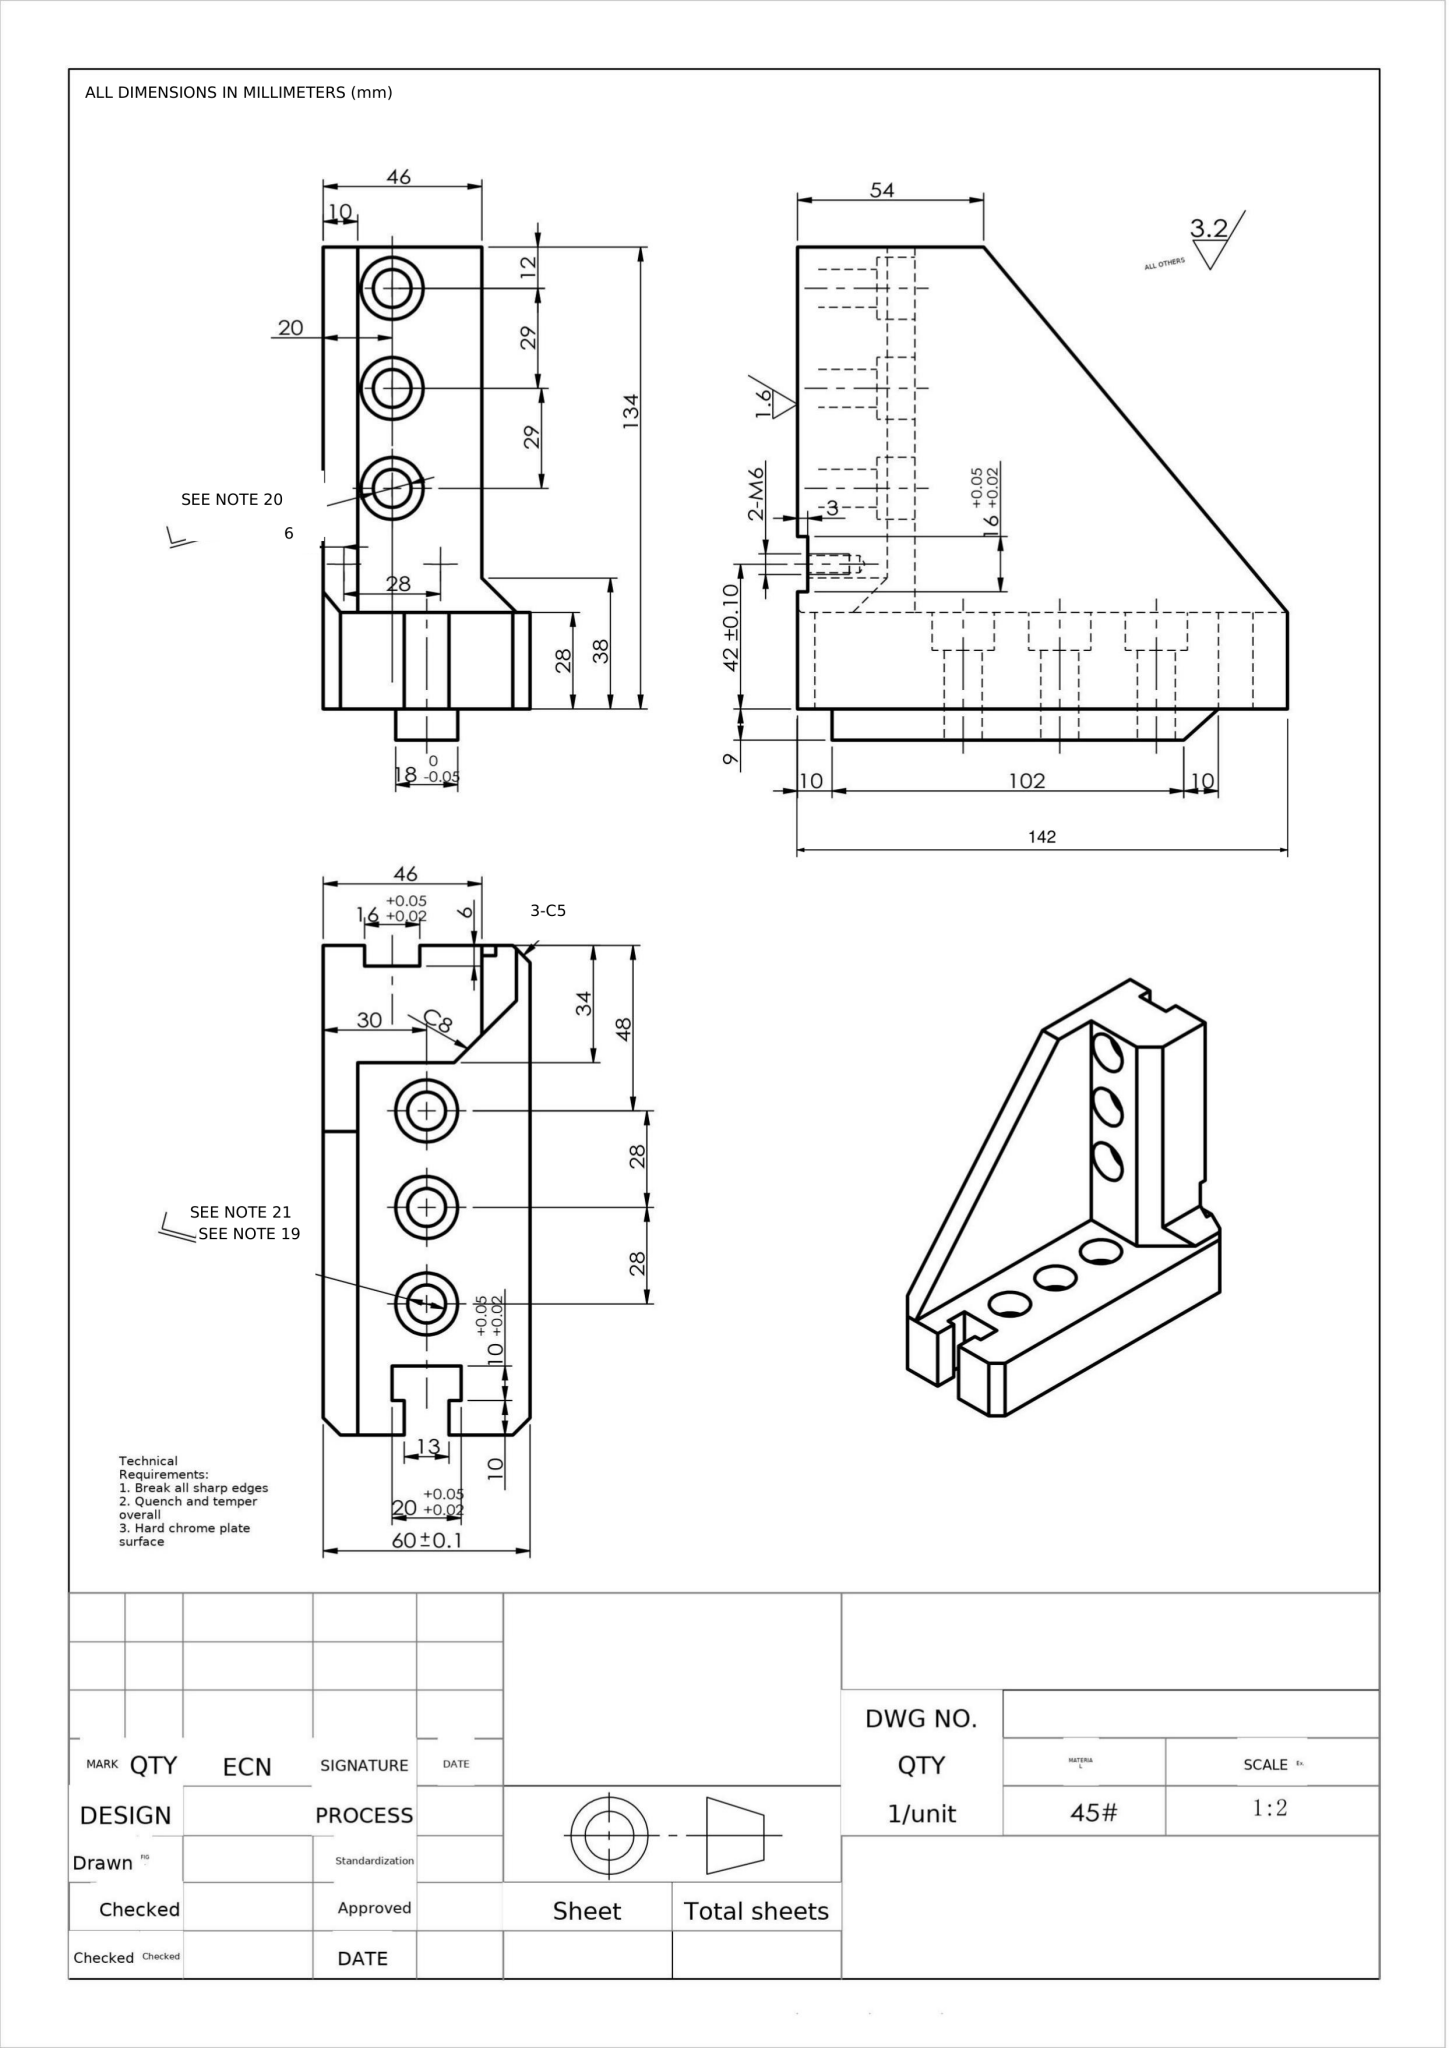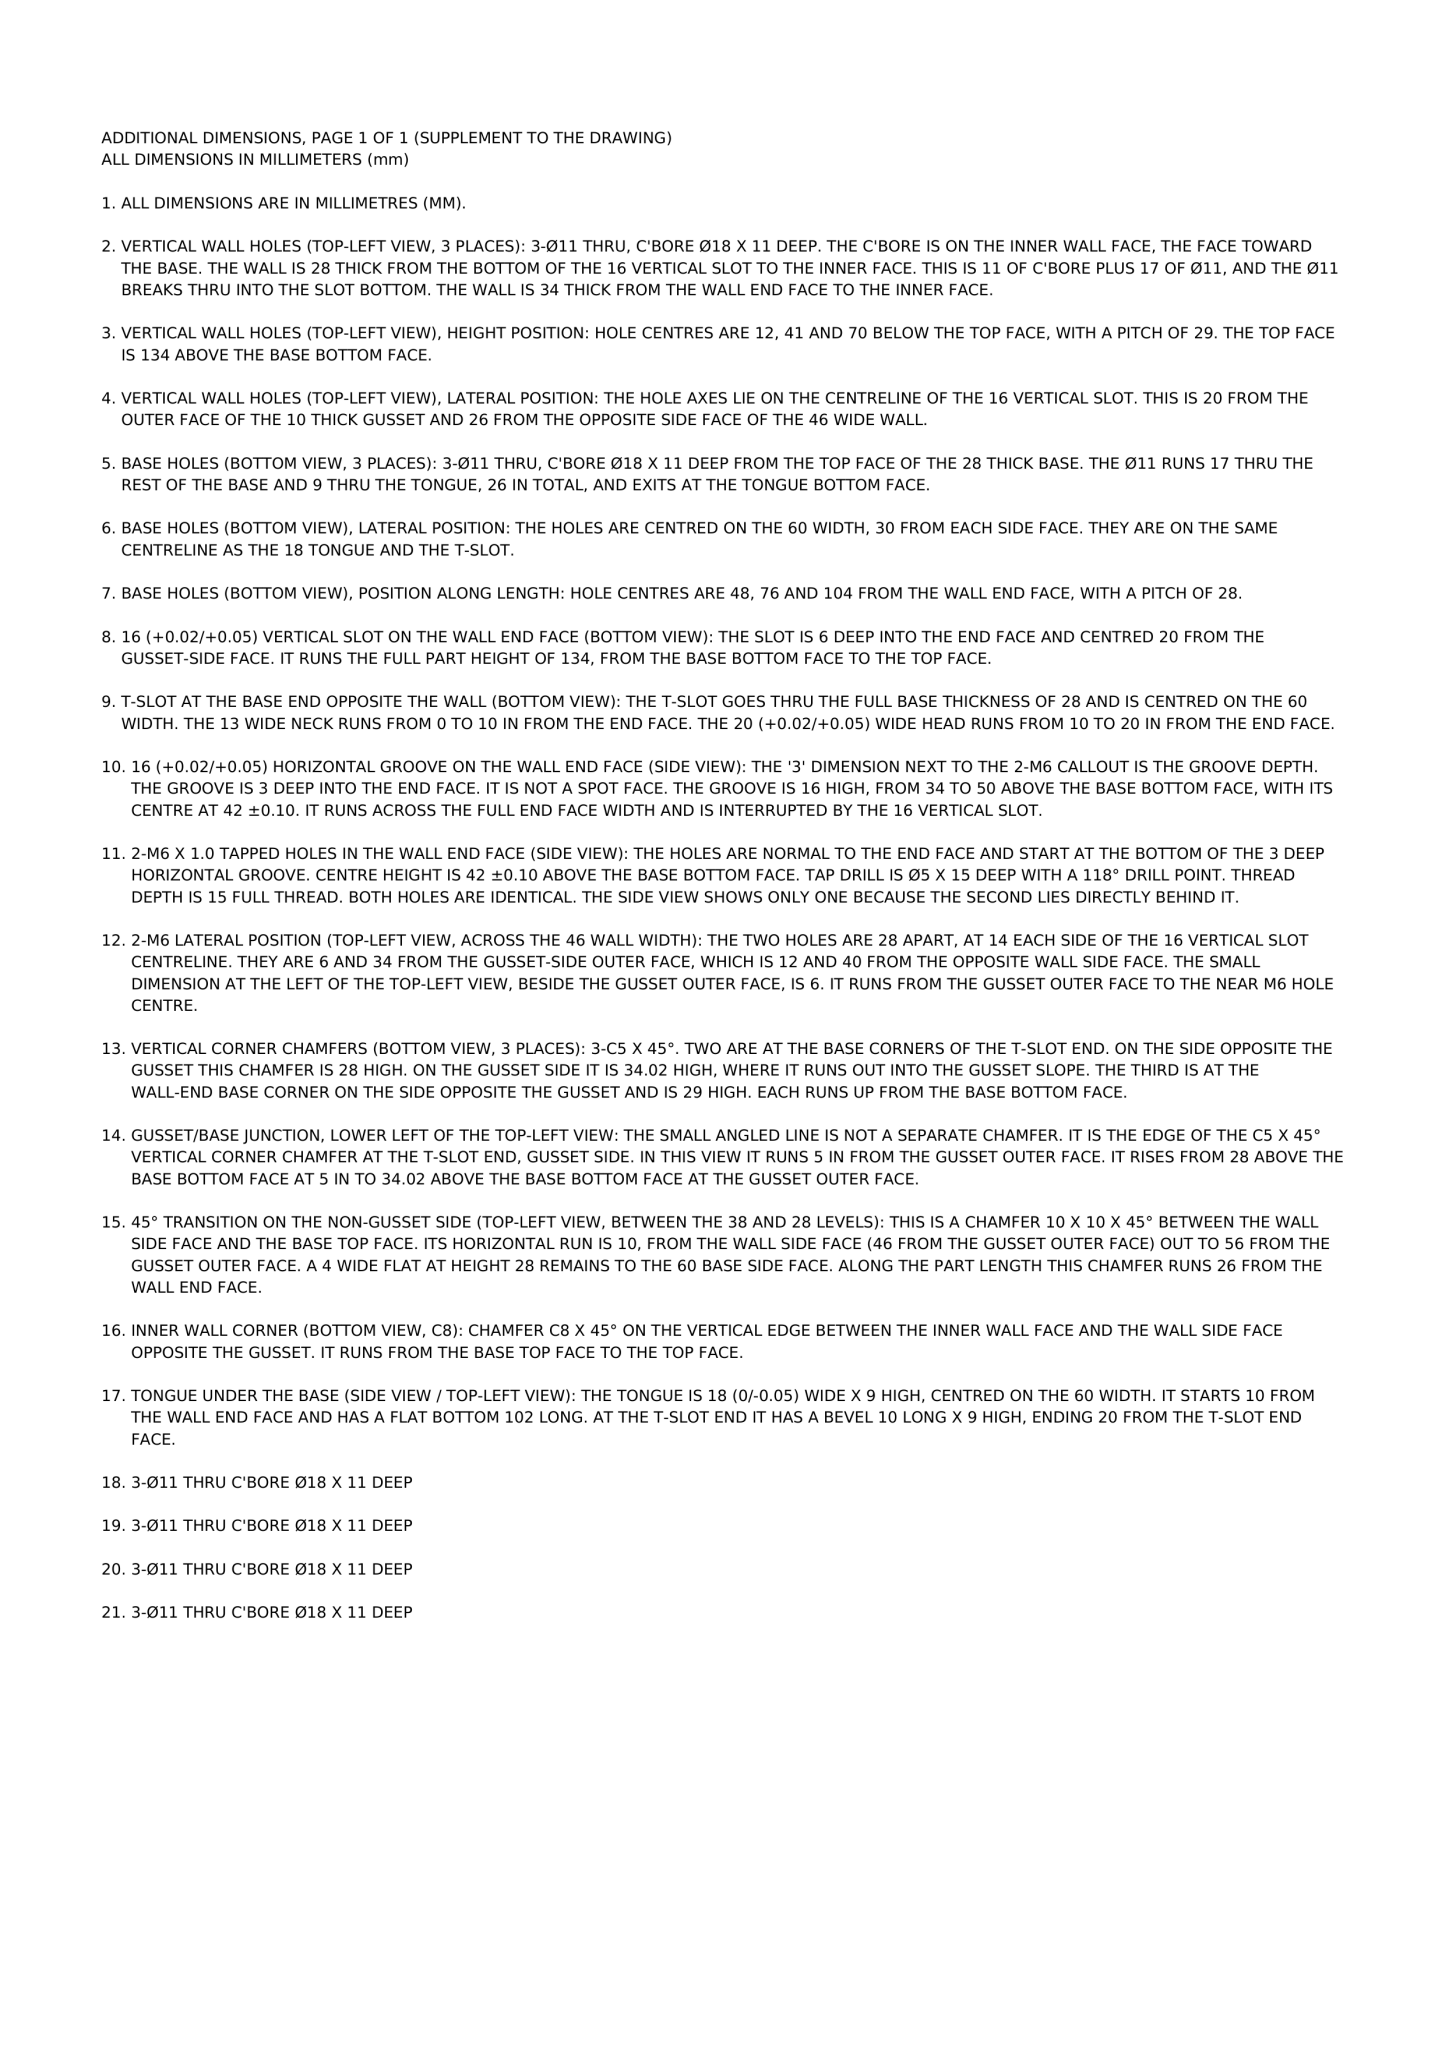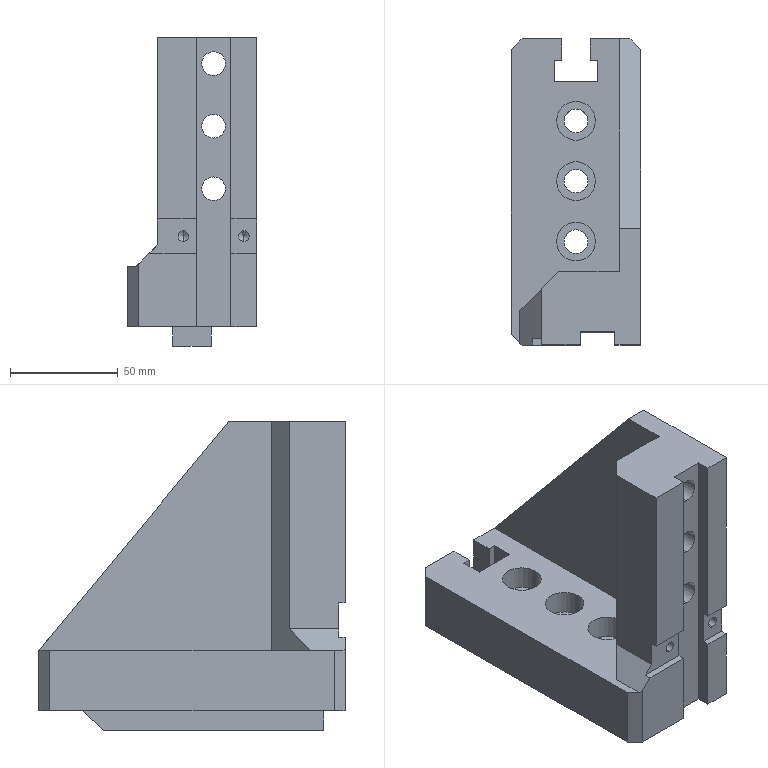Part | NX | mm | 1 solid | 79 faces | box 60 x 142 x 143 mm | volume 432953 mm3 | plane 47 | cylinder 28 | cone 4 | commonest cylinder face diameters 18 x12 11 x12 5 x4